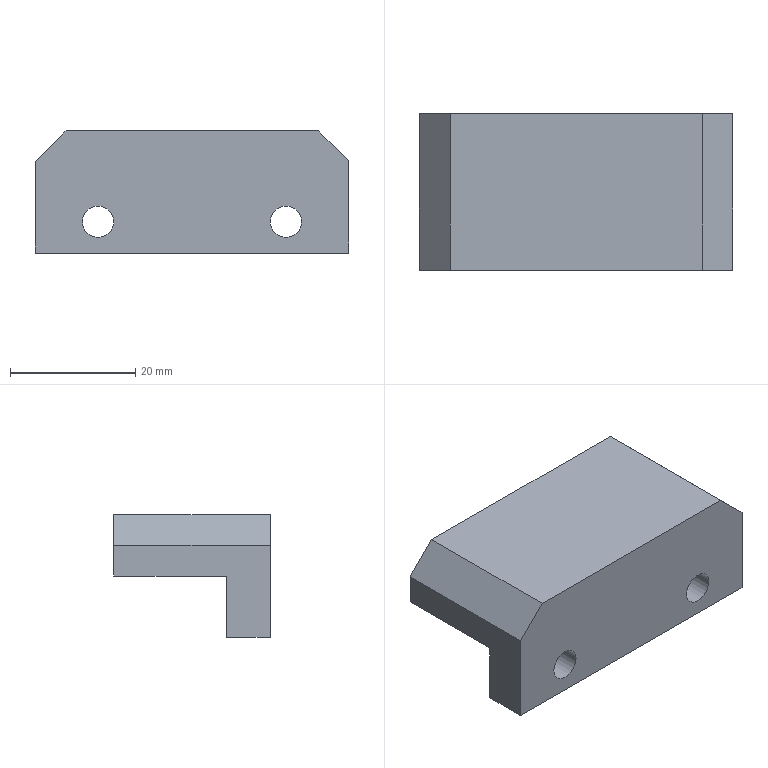Component | SolidWorks | LegSupport-1 | 1 solid | 22 faces | box 50 x 25 x 19.5 mm | volume 14508 mm3 | plane 10 | cylinder 8 | cone 4 | commonest cylinder face diameters 5 x4 2.5 x4
build123d program:
from build123d import *

# Parameters (mm, degrees)
SKETCH2_W             = 17
SKETCH2_H             = 50
BOSS_EXTRUDE1_DEPTH   = 25
M3_TAPPED_HOLE1_D     = 2.5
M3_TAPPED_HOLE1_DEPTH = 12.5
M3_TAPPED_HOLE1_TIP   = 0.7511
SKETCH5_W             = 10
SKETCH5_H             = 50
BOSS_EXTRUDE2_DEPTH   = 25
CUT_EXTRUDE1_DEPTH    = 18
SKETCH7_R             = 2.5
CUT_EXTRUDE2_DEPTH    = 38.027
CUT_EXTRUDE3_REACH    = 39.027


with BuildPart() as part:
    # Sketch2 → Boss-Extrude1 (new body)
    with BuildSketch(Plane(origin=(0, 0, 0), x_dir=(1, 0, 0), z_dir=(0, 1, 0))):
        Rectangle(SKETCH2_W, SKETCH2_H)
    extrude(amount=BOSS_EXTRUDE1_DEPTH)

    # M3 Tapped Hole1
    with Locations(Plane(origin=(6, 25, -15), x_dir=(0, 0, 1), z_dir=(0, 1, 0))):
        with Locations((0, 0), (30, 0)):
            Hole(M3_TAPPED_HOLE1_D / 2, depth=M3_TAPPED_HOLE1_DEPTH)
            with Locations((0, 0, -(M3_TAPPED_HOLE1_DEPTH + M3_TAPPED_HOLE1_TIP / 2))):  # 118° drill point
                Cone(0, M3_TAPPED_HOLE1_D / 2, M3_TAPPED_HOLE1_TIP, mode=Mode.SUBTRACT)

    # Sketch5 → Boss-Extrude2 (add)
    with BuildSketch(Plane(origin=(0, 25, 0), x_dir=(1, 0, 0), z_dir=(0, 1, 0))):
        with Locations((-6, 0)):
            Rectangle(SKETCH5_W, SKETCH5_H)
    extrude(amount=-BOSS_EXTRUDE2_DEPTH)

    # Sketch6 → Cut-Extrude1 (cut)
    with BuildSketch(Plane(origin=(0, 25, 0), x_dir=(1, 0, 0), z_dir=(0, 1, 0))):
        Polygon((-11, 25), (-1, 25), (-1.25, -25), (-11, -25), align=None)
    extrude(amount=-CUT_EXTRUDE1_DEPTH, mode=Mode.SUBTRACT)

    # Sketch7 → Cut-Extrude2 (cut, through all)
    with BuildSketch(Plane(origin=(0, 25, 0), x_dir=(1, 0, 0), z_dir=(0, 1, 0))):
        with Locations(Location((-6, 15, 0), (0, 0, 270))):
            Circle(SKETCH7_R)
        with Locations(Location((-6, -15, 0), (0, 0, 270))):
            Circle(SKETCH7_R)
    extrude(amount=-CUT_EXTRUDE2_DEPTH, mode=Mode.SUBTRACT)

    # Sketch8 → Cut-Extrude3 (cut, up to next)
    with BuildSketch(Plane(origin=(0, 25, 0), x_dir=(1, 0, 0), z_dir=(0, 1, 0)), mode=Mode.PRIVATE) as cut_extrude3_sk1:
        Polygon((8.5, 25), (3.75, 25), (8.5, 20.25), align=None)
    cut_extrude3_tool1 = extrude(cut_extrude3_sk1.sketch, amount=-CUT_EXTRUDE3_REACH, mode=Mode.PRIVATE) & part.part
    # Sketch8 → Cut-Extrude3 (cut, up to next)
    with BuildSketch(Plane(origin=(0, 25, 0), x_dir=(1, 0, 0), z_dir=(0, 1, 0)), mode=Mode.PRIVATE) as cut_extrude3_sk2:
        Polygon((8.5, -25), (8.5, -20.125), (3.625, -25), align=None)
    cut_extrude3_tool2 = extrude(cut_extrude3_sk2.sketch, amount=-CUT_EXTRUDE3_REACH, mode=Mode.PRIVATE) & part.part
    add(cut_extrude3_tool1.solids().sort_by_distance((6.917, 25, -23.417))[0], mode=Mode.SUBTRACT)
    add(cut_extrude3_tool2.solids().sort_by_distance((6.875, 25, 23.375))[0], mode=Mode.SUBTRACT)


solid = part.part

# Placed as in the assembly
solid = solid.moved(Location((-24.154, 53.266, -195.507), (0, -90, 0)))
STEP:
#1=CARTESIAN_POINT('',(-1.443,2.097,-7.933));
#2=VERTEX_POINT('',#1);
#3=CARTESIAN_POINT('',(-1.64,2.097,-7.933));
#4=VERTEX_POINT('',#3);
#5=CARTESIAN_POINT('',(-1.542,2.097,-7.933));
#6=DIRECTION('',(0.,1.,0.));
#7=DIRECTION('',(-1.,0.,0.));
#8=AXIS2_PLACEMENT_3D('',#5,#6,#7);
#9=CIRCLE('',#8,0.09843);
#10=EDGE_CURVE('',#2,#4,#9,.T.);
#11=ORIENTED_EDGE('',*,*,#10,.F.);
#12=CARTESIAN_POINT('',(-1.443,2.373,-7.933));
#13=VERTEX_POINT('',#12);
#14=CARTESIAN_POINT('',(-1.443,2.097,-7.933));
#15=DIRECTION('',(0.,1.,0.));
#16=VECTOR('',#15,39.37);
#17=LINE('',#14,#16);
#18=EDGE_CURVE('',#2,#13,#17,.T.);
#19=ORIENTED_EDGE('',*,*,#18,.T.);
#20=CARTESIAN_POINT('',(-1.64,2.373,-7.933));
#21=VERTEX_POINT('',#20);
#22=CARTESIAN_POINT('',(-1.542,2.373,-7.933));
#23=DIRECTION('',(0.,1.,0.));
#24=DIRECTION('',(-1.,0.,0.));
#25=AXIS2_PLACEMENT_3D('',#22,#23,#24);
#26=CIRCLE('',#25,0.09843);
#27=EDGE_CURVE('',#13,#21,#26,.T.);
#28=ORIENTED_EDGE('',*,*,#27,.T.);
#29=CARTESIAN_POINT('',(-1.64,2.097,-7.933));
#30=DIRECTION('',(0.,1.,0.));
#31=VECTOR('',#30,39.37);
#32=LINE('',#29,#31);
#33=EDGE_CURVE('',#4,#21,#32,.T.);
#34=ORIENTED_EDGE('',*,*,#33,.F.);
#35=EDGE_LOOP('',(#11,#19,#28,#34));
#36=FACE_OUTER_BOUND('',#35,.T.);
#37=CARTESIAN_POINT('',(-1.542,2.097,-7.933));
#38=DIRECTION('',(0.,1.,0.));
#39=DIRECTION('',(-1.,0.,0.));
#40=AXIS2_PLACEMENT_3D('',#37,#38,#39);
#41=CYLINDRICAL_SURFACE('',#40,0.09843);
#42=ADVANCED_FACE('',(#36),#41,.F.);
#43=CARTESIAN_POINT('',(-0.262,2.097,-7.933));
#44=VERTEX_POINT('',#43);
#45=CARTESIAN_POINT('',(-0.4588,2.097,-7.933));
#46=VERTEX_POINT('',#45);
#47=CARTESIAN_POINT('',(-0.3604,2.097,-7.933));
#48=DIRECTION('',(0.,1.,0.));
#49=DIRECTION('',(-1.,0.,0.));
#50=AXIS2_PLACEMENT_3D('',#47,#48,#49);
#51=CIRCLE('',#50,0.09843);
#52=EDGE_CURVE('',#44,#46,#51,.T.);
#53=ORIENTED_EDGE('',*,*,#52,.F.);
#54=CARTESIAN_POINT('',(-0.262,2.373,-7.933));
#55=VERTEX_POINT('',#54);
#56=CARTESIAN_POINT('',(-0.262,2.097,-7.933));
#57=DIRECTION('',(0.,1.,0.));
#58=VECTOR('',#57,39.37);
#59=LINE('',#56,#58);
#60=EDGE_CURVE('',#44,#55,#59,.T.);
#61=ORIENTED_EDGE('',*,*,#60,.T.);
#62=CARTESIAN_POINT('',(-0.4588,2.373,-7.933));
#63=VERTEX_POINT('',#62);
#64=CARTESIAN_POINT('',(-0.3604,2.373,-7.933));
#65=DIRECTION('',(0.,1.,0.));
#66=DIRECTION('',(-1.,0.,0.));
#67=AXIS2_PLACEMENT_3D('',#64,#65,#66);
#68=CIRCLE('',#67,0.09843);
#69=EDGE_CURVE('',#55,#63,#68,.T.);
#70=ORIENTED_EDGE('',*,*,#69,.T.);
#71=CARTESIAN_POINT('',(-0.4588,2.097,-7.933));
#72=DIRECTION('',(0.,1.,0.));
#73=VECTOR('',#72,39.37);
#74=LINE('',#71,#73);
#75=EDGE_CURVE('',#46,#63,#74,.T.);
#76=ORIENTED_EDGE('',*,*,#75,.F.);
#77=EDGE_LOOP('',(#53,#61,#70,#76));
#78=FACE_OUTER_BOUND('',#77,.T.);
#79=CARTESIAN_POINT('',(-0.3604,2.097,-7.933));
#80=DIRECTION('',(0.,1.,0.));
#81=DIRECTION('',(-1.,0.,0.));
#82=AXIS2_PLACEMENT_3D('',#79,#80,#81);
#83=CYLINDRICAL_SURFACE('',#82,0.09843);
#84=ADVANCED_FACE('',(#78),#83,.F.);
#85=CARTESIAN_POINT('',(-0.3112,2.589,-7.461));
#86=VERTEX_POINT('',#85);
#87=CARTESIAN_POINT('',(-0.4096,2.589,-7.461));
#88=VERTEX_POINT('',#87);
#89=CARTESIAN_POINT('',(-0.3604,2.589,-7.461));
#90=DIRECTION('',(0.,1.,0.));
#91=DIRECTION('',(-1.,0.,0.));
#92=AXIS2_PLACEMENT_3D('',#89,#90,#91);
#93=CIRCLE('',#92,0.04921);
#94=EDGE_CURVE('',#86,#88,#93,.T.);
#95=ORIENTED_EDGE('',*,*,#94,.F.);
#96=CARTESIAN_POINT('',(-0.3112,3.081,-7.461));
#97=VERTEX_POINT('',#96);
#98=CARTESIAN_POINT('',(-0.3112,3.081,-7.461));
#99=DIRECTION('',(0.,1.,0.));
#100=VECTOR('',#99,39.37);
#101=LINE('',#98,#100);
#102=EDGE_CURVE('',#86,#97,#101,.T.);
#103=ORIENTED_EDGE('',*,*,#102,.T.);
#104=CARTESIAN_POINT('',(-0.4096,3.081,-7.461));
#105=VERTEX_POINT('',#104);
#106=CARTESIAN_POINT('',(-0.3604,3.081,-7.461));
#107=DIRECTION('',(0.,1.,0.));
#108=DIRECTION('',(-1.,0.,0.));
#109=AXIS2_PLACEMENT_3D('',#106,#107,#108);
#110=CIRCLE('',#109,0.04921);
#111=EDGE_CURVE('',#97,#105,#110,.T.);
#112=ORIENTED_EDGE('',*,*,#111,.T.);
#113=CARTESIAN_POINT('',(-0.4096,3.081,-7.461));
#114=DIRECTION('',(0.,1.,0.));
#115=VECTOR('',#114,39.37);
#116=LINE('',#113,#115);
#117=EDGE_CURVE('',#88,#105,#116,.T.);
#118=ORIENTED_EDGE('',*,*,#117,.F.);
#119=EDGE_LOOP('',(#95,#103,#112,#118));
#120=FACE_OUTER_BOUND('',#119,.T.);
#121=CARTESIAN_POINT('',(-0.3604,3.081,-7.461));
#122=DIRECTION('',(0.,1.,0.));
#123=DIRECTION('',(-1.,0.,0.));
#124=AXIS2_PLACEMENT_3D('',#121,#122,#123);
#125=CYLINDRICAL_SURFACE('',#124,0.04921);
#126=ADVANCED_FACE('',(#120),#125,.F.);
#127=CARTESIAN_POINT('',(-0.3604,2.56,-7.461));
#128=VERTEX_POINT('',#127);
#129=CARTESIAN_POINT('',(-0.4096,2.589,-7.461));
#130=DIRECTION('',(-0.8572,0.515,-0.));
#131=VECTOR('',#130,39.37);
#132=LINE('',#129,#131);
#133=EDGE_CURVE('',#128,#88,#132,.T.);
#134=ORIENTED_EDGE('',*,*,#133,.F.);
#135=CARTESIAN_POINT('',(-0.3112,2.589,-7.461));
#136=DIRECTION('',(0.8572,0.515,0.));
#137=VECTOR('',#136,39.37);
#138=LINE('',#135,#137);
#139=EDGE_CURVE('',#128,#86,#138,.T.);
#140=ORIENTED_EDGE('',*,*,#139,.T.);
#141=ORIENTED_EDGE('',*,*,#94,.T.);
#142=EDGE_LOOP('',(#134,#140,#141));
#143=FACE_OUTER_BOUND('',#142,.T.);
#144=CARTESIAN_POINT('',(-0.3604,2.589,-7.461));
#145=DIRECTION('',(0.,1.,0.));
#146=DIRECTION('',(-1.,0.,0.));
#147=AXIS2_PLACEMENT_3D('',#144,#145,#146);
#148=CONICAL_SURFACE('',#147,0.04921,1.03);
#149=ADVANCED_FACE('',(#143),#148,.F.);
#150=CARTESIAN_POINT('',(-1.492,2.589,-7.461));
#151=VERTEX_POINT('',#150);
#152=CARTESIAN_POINT('',(-1.591,2.589,-7.461));
#153=VERTEX_POINT('',#152);
#154=CARTESIAN_POINT('',(-1.542,2.589,-7.461));
#155=DIRECTION('',(0.,1.,0.));
#156=DIRECTION('',(-1.,0.,0.));
#157=AXIS2_PLACEMENT_3D('',#154,#155,#156);
#158=CIRCLE('',#157,0.04921);
#159=EDGE_CURVE('',#151,#153,#158,.T.);
#160=ORIENTED_EDGE('',*,*,#159,.F.);
#161=CARTESIAN_POINT('',(-1.492,3.081,-7.461));
#162=VERTEX_POINT('',#161);
#163=CARTESIAN_POINT('',(-1.492,3.081,-7.461));
#164=DIRECTION('',(0.,1.,0.));
#165=VECTOR('',#164,39.37);
#166=LINE('',#163,#165);
#167=EDGE_CURVE('',#151,#162,#166,.T.);
#168=ORIENTED_EDGE('',*,*,#167,.T.);
#169=CARTESIAN_POINT('',(-1.591,3.081,-7.461));
#170=VERTEX_POINT('',#169);
#171=CARTESIAN_POINT('',(-1.542,3.081,-7.461));
#172=DIRECTION('',(0.,1.,0.));
#173=DIRECTION('',(-1.,0.,0.));
#174=AXIS2_PLACEMENT_3D('',#171,#172,#173);
#175=CIRCLE('',#174,0.04921);
#176=EDGE_CURVE('',#162,#170,#175,.T.);
#177=ORIENTED_EDGE('',*,*,#176,.T.);
#178=CARTESIAN_POINT('',(-1.591,3.081,-7.461));
#179=DIRECTION('',(0.,1.,0.));
#180=VECTOR('',#179,39.37);
#181=LINE('',#178,#180);
#182=EDGE_CURVE('',#153,#170,#181,.T.);
#183=ORIENTED_EDGE('',*,*,#182,.F.);
#184=EDGE_LOOP('',(#160,#168,#177,#183));
#185=FACE_OUTER_BOUND('',#184,.T.);
#186=CARTESIAN_POINT('',(-1.542,3.081,-7.461));
#187=DIRECTION('',(0.,1.,0.));
#188=DIRECTION('',(-1.,0.,0.));
#189=AXIS2_PLACEMENT_3D('',#186,#187,#188);
#190=CYLINDRICAL_SURFACE('',#189,0.04921);
#191=ADVANCED_FACE('',(#185),#190,.F.);
#192=CARTESIAN_POINT('',(-1.542,2.56,-7.461));
#193=VERTEX_POINT('',#192);
#194=CARTESIAN_POINT('',(-1.591,2.589,-7.461));
#195=DIRECTION('',(-0.8572,0.515,-0.));
#196=VECTOR('',#195,39.37);
#197=LINE('',#194,#196);
#198=EDGE_CURVE('',#193,#153,#197,.T.);
#199=ORIENTED_EDGE('',*,*,#198,.F.);
#200=CARTESIAN_POINT('',(-1.492,2.589,-7.461));
#201=DIRECTION('',(0.8572,0.515,0.));
#202=VECTOR('',#201,39.37);
#203=LINE('',#200,#202);
#204=EDGE_CURVE('',#193,#151,#203,.T.);
#205=ORIENTED_EDGE('',*,*,#204,.T.);
#206=ORIENTED_EDGE('',*,*,#159,.T.);
#207=EDGE_LOOP('',(#199,#205,#206));
#208=FACE_OUTER_BOUND('',#207,.T.);
#209=CARTESIAN_POINT('',(-1.542,2.589,-7.461));
#210=DIRECTION('',(0.,1.,0.));
#211=DIRECTION('',(-1.,0.,0.));
#212=AXIS2_PLACEMENT_3D('',#209,#210,#211);
#213=CONICAL_SURFACE('',#212,0.04921,1.03);
#214=ADVANCED_FACE('',(#208),#213,.F.);
#215=CARTESIAN_POINT('',(-1.743,2.097,-7.362));
#216=VERTEX_POINT('',#215);
#217=CARTESIAN_POINT('',(-1.743,3.081,-7.362));
#218=VERTEX_POINT('',#217);
#219=CARTESIAN_POINT('',(-1.743,2.097,-7.362));
#220=DIRECTION('',(0.,1.,0.));
#221=VECTOR('',#220,39.37);
#222=LINE('',#219,#221);
#223=EDGE_CURVE('',#216,#218,#222,.T.);
#224=ORIENTED_EDGE('',*,*,#223,.F.);
#225=CARTESIAN_POINT('',(-0.1537,2.097,-7.362));
#226=VERTEX_POINT('',#225);
#227=CARTESIAN_POINT('',(0.03329,2.097,-7.362));
#228=DIRECTION('',(1.,0.,0.));
#229=VECTOR('',#228,39.37);
#230=LINE('',#227,#229);
#231=EDGE_CURVE('',#216,#226,#230,.T.);
#232=ORIENTED_EDGE('',*,*,#231,.T.);
#233=CARTESIAN_POINT('',(-0.1537,3.081,-7.362));
#234=VERTEX_POINT('',#233);
#235=CARTESIAN_POINT('',(-0.1537,2.097,-7.362));
#236=DIRECTION('',(0.,1.,0.));
#237=VECTOR('',#236,39.37);
#238=LINE('',#235,#237);
#239=EDGE_CURVE('',#226,#234,#238,.T.);
#240=ORIENTED_EDGE('',*,*,#239,.T.);
#241=CARTESIAN_POINT('',(0.03329,3.081,-7.362));
#242=DIRECTION('',(1.,0.,0.));
#243=VECTOR('',#242,39.37);
#244=LINE('',#241,#243);
#245=EDGE_CURVE('',#218,#234,#244,.T.);
#246=ORIENTED_EDGE('',*,*,#245,.F.);
#247=EDGE_LOOP('',(#224,#232,#240,#246));
#248=FACE_OUTER_BOUND('',#247,.T.);
#249=CARTESIAN_POINT('',(0.03329,3.081,-7.362));
#250=DIRECTION('',(0.,0.,-1.));
#251=DIRECTION('',(-1.,0.,-0.));
#252=AXIS2_PLACEMENT_3D('',#249,#250,#251);
#253=PLANE('',#252);
#254=ADVANCED_FACE('',(#248),#253,.F.);
#255=CARTESIAN_POINT('',(-1.935,2.097,-7.554));
#256=VERTEX_POINT('',#255);
#257=CARTESIAN_POINT('',(-1.935,3.081,-7.554));
#258=VERTEX_POINT('',#257);
#259=CARTESIAN_POINT('',(-1.935,2.097,-7.554));
#260=DIRECTION('',(0.,1.,0.));
#261=VECTOR('',#260,39.37);
#262=LINE('',#259,#261);
#263=EDGE_CURVE('',#256,#258,#262,.T.);
#264=ORIENTED_EDGE('',*,*,#263,.T.);
#265=CARTESIAN_POINT('',(-1.935,3.081,-7.746));
#266=VERTEX_POINT('',#265);
#267=CARTESIAN_POINT('',(-1.935,3.081,-8.032));
#268=DIRECTION('',(-0.,0.,1.));
#269=VECTOR('',#268,39.37);
#270=LINE('',#267,#269);
#271=EDGE_CURVE('',#266,#258,#270,.T.);
#272=ORIENTED_EDGE('',*,*,#271,.F.);
#273=CARTESIAN_POINT('',(-1.935,2.373,-7.746));
#274=VERTEX_POINT('',#273);
#275=CARTESIAN_POINT('',(-1.935,2.373,-7.746));
#276=DIRECTION('',(0.,1.,0.));
#277=VECTOR('',#276,39.37);
#278=LINE('',#275,#277);
#279=EDGE_CURVE('',#274,#266,#278,.T.);
#280=ORIENTED_EDGE('',*,*,#279,.F.);
#281=CARTESIAN_POINT('',(-1.935,2.373,-8.13));
#282=VERTEX_POINT('',#281);
#283=CARTESIAN_POINT('',(-1.935,2.373,-8.13));
#284=DIRECTION('',(0.,0.,1.));
#285=VECTOR('',#284,39.37);
#286=LINE('',#283,#285);
#287=EDGE_CURVE('',#282,#274,#286,.T.);
#288=ORIENTED_EDGE('',*,*,#287,.F.);
#289=CARTESIAN_POINT('',(-1.935,2.097,-8.13));
#290=VERTEX_POINT('',#289);
#291=CARTESIAN_POINT('',(-1.935,2.097,-8.13));
#292=DIRECTION('',(0.,1.,0.));
#293=VECTOR('',#292,39.37);
#294=LINE('',#291,#293);
#295=EDGE_CURVE('',#290,#282,#294,.T.);
#296=ORIENTED_EDGE('',*,*,#295,.F.);
#297=CARTESIAN_POINT('',(-1.935,2.097,-8.032));
#298=DIRECTION('',(-0.,0.,1.));
#299=VECTOR('',#298,39.37);
#300=LINE('',#297,#299);
#301=EDGE_CURVE('',#290,#256,#300,.T.);
#302=ORIENTED_EDGE('',*,*,#301,.T.);
#303=EDGE_LOOP('',(#264,#272,#280,#288,#296,#302));
#304=FACE_OUTER_BOUND('',#303,.T.);
#305=CARTESIAN_POINT('',(-1.935,3.081,-8.032));
#306=DIRECTION('',(1.,0.,0.));
#307=DIRECTION('',(0.,0.,-1.));
#308=AXIS2_PLACEMENT_3D('',#305,#306,#307);
#309=PLANE('',#308);
#310=ADVANCED_FACE('',(#304),#309,.F.);
#311=CARTESIAN_POINT('',(-0.3604,3.081,-7.461));
#312=DIRECTION('',(0.,1.,0.));
#313=DIRECTION('',(-1.,0.,0.));
#314=AXIS2_PLACEMENT_3D('',#311,#312,#313);
#315=CIRCLE('',#314,0.04921);
#316=EDGE_CURVE('',#105,#97,#315,.T.);
#317=ORIENTED_EDGE('',*,*,#316,.F.);
#318=ORIENTED_EDGE('',*,*,#111,.F.);
#319=EDGE_LOOP('',(#317,#318));
#320=FACE_BOUND('',#319,.T.);
#321=CARTESIAN_POINT('',(-1.542,3.081,-7.461));
#322=DIRECTION('',(0.,1.,0.));
#323=DIRECTION('',(-1.,0.,0.));
#324=AXIS2_PLACEMENT_3D('',#321,#322,#323);
#325=CIRCLE('',#324,0.04921);
#326=EDGE_CURVE('',#170,#162,#325,.T.);
#327=ORIENTED_EDGE('',*,*,#326,.F.);
#328=ORIENTED_EDGE('',*,*,#176,.F.);
#329=EDGE_LOOP('',(#327,#328));
#330=FACE_BOUND('',#329,.T.);
#331=ORIENTED_EDGE('',*,*,#271,.T.);
#332=CARTESIAN_POINT('',(-1.514,3.081,-7.134));
#333=DIRECTION('',(0.7071,0.,0.7071));
#334=VECTOR('',#333,39.37);
#335=LINE('',#332,#334);
#336=EDGE_CURVE('',#258,#218,#335,.T.);
#337=ORIENTED_EDGE('',*,*,#336,.T.);
#338=ORIENTED_EDGE('',*,*,#245,.T.);
#339=CARTESIAN_POINT('',(0.03329,3.081,-7.549));
#340=VERTEX_POINT('',#339);
#341=CARTESIAN_POINT('',(-0.385,3.081,-7.131));
#342=DIRECTION('',(-0.7071,0.,0.7071));
#343=VECTOR('',#342,39.37);
#344=LINE('',#341,#343);
#345=EDGE_CURVE('',#340,#234,#344,.T.);
#346=ORIENTED_EDGE('',*,*,#345,.F.);
#347=CARTESIAN_POINT('',(0.03329,3.081,-7.736));
#348=VERTEX_POINT('',#347);
#349=CARTESIAN_POINT('',(0.03329,3.081,-8.032));
#350=DIRECTION('',(0.,0.,-1.));
#351=VECTOR('',#350,39.37);
#352=LINE('',#349,#351);
#353=EDGE_CURVE('',#340,#348,#352,.T.);
#354=ORIENTED_EDGE('',*,*,#353,.T.);
#355=CARTESIAN_POINT('',(0.03329,3.081,-7.736));
#356=DIRECTION('',(1.,0.,0.005));
#357=VECTOR('',#356,39.37);
#358=LINE('',#355,#357);
#359=EDGE_CURVE('',#266,#348,#358,.T.);
#360=ORIENTED_EDGE('',*,*,#359,.F.);
#361=EDGE_LOOP('',(#331,#337,#338,#346,#354,#360));
#362=FACE_OUTER_BOUND('',#361,.T.);
#363=CARTESIAN_POINT('',(-0.951,3.081,-7.697));
#364=DIRECTION('',(0.,1.,0.));
#365=DIRECTION('',(-1.,0.,-0.));
#366=AXIS2_PLACEMENT_3D('',#363,#364,#365);
#367=PLANE('',#366);
#368=ADVANCED_FACE('',(#320,#330,#362),#367,.T.);
#369=CARTESIAN_POINT('',(-0.3604,2.097,-7.933));
#370=DIRECTION('',(0.,1.,0.));
#371=DIRECTION('',(-1.,0.,0.));
#372=AXIS2_PLACEMENT_3D('',#369,#370,#371);
#373=CIRCLE('',#372,0.09843);
#374=EDGE_CURVE('',#46,#44,#373,.T.);
#375=ORIENTED_EDGE('',*,*,#374,.T.);
#376=ORIENTED_EDGE('',*,*,#52,.T.);
#377=EDGE_LOOP('',(#375,#376));
#378=FACE_BOUND('',#377,.T.);
#379=CARTESIAN_POINT('',(-1.542,2.097,-7.933));
#380=DIRECTION('',(0.,1.,0.));
#381=DIRECTION('',(-1.,0.,0.));
#382=AXIS2_PLACEMENT_3D('',#379,#380,#381);
#383=CIRCLE('',#382,0.09843);
#384=EDGE_CURVE('',#4,#2,#383,.T.);
#385=ORIENTED_EDGE('',*,*,#384,.T.);
#386=ORIENTED_EDGE('',*,*,#10,.T.);
#387=EDGE_LOOP('',(#385,#386));
#388=FACE_BOUND('',#387,.T.);
#389=CARTESIAN_POINT('',(-1.514,2.097,-7.134));
#390=DIRECTION('',(-0.7071,0.,-0.7071));
#391=VECTOR('',#390,39.37);
#392=LINE('',#389,#391);
#393=EDGE_CURVE('',#216,#256,#392,.T.);
#394=ORIENTED_EDGE('',*,*,#393,.T.);
#395=ORIENTED_EDGE('',*,*,#301,.F.);
#396=CARTESIAN_POINT('',(0.03329,2.097,-8.13));
#397=VERTEX_POINT('',#396);
#398=CARTESIAN_POINT('',(0.03329,2.097,-8.13));
#399=DIRECTION('',(-1.,0.,-0.));
#400=VECTOR('',#399,39.37);
#401=LINE('',#398,#400);
#402=EDGE_CURVE('',#397,#290,#401,.T.);
#403=ORIENTED_EDGE('',*,*,#402,.F.);
#404=CARTESIAN_POINT('',(0.03329,2.097,-7.549));
#405=VERTEX_POINT('',#404);
#406=CARTESIAN_POINT('',(0.03329,2.097,-8.032));
#407=DIRECTION('',(0.,0.,-1.));
#408=VECTOR('',#407,39.37);
#409=LINE('',#406,#408);
#410=EDGE_CURVE('',#405,#397,#409,.T.);
#411=ORIENTED_EDGE('',*,*,#410,.F.);
#412=CARTESIAN_POINT('',(-0.385,2.097,-7.131));
#413=DIRECTION('',(0.7071,0.,-0.7071));
#414=VECTOR('',#413,39.37);
#415=LINE('',#412,#414);
#416=EDGE_CURVE('',#226,#405,#415,.T.);
#417=ORIENTED_EDGE('',*,*,#416,.F.);
#418=ORIENTED_EDGE('',*,*,#231,.F.);
#419=EDGE_LOOP('',(#394,#395,#403,#411,#417,#418));
#420=FACE_OUTER_BOUND('',#419,.T.);
#421=CARTESIAN_POINT('',(-0.951,2.097,-7.697));
#422=DIRECTION('',(0.,1.,0.));
#423=DIRECTION('',(-1.,0.,-0.));
#424=AXIS2_PLACEMENT_3D('',#421,#422,#423);
#425=PLANE('',#424);
#426=ADVANCED_FACE('',(#378,#388,#420),#425,.F.);
#427=ORIENTED_EDGE('',*,*,#295,.T.);
#428=CARTESIAN_POINT('',(0.03329,2.373,-8.13));
#429=VERTEX_POINT('',#428);
#430=CARTESIAN_POINT('',(0.03329,2.373,-8.13));
#431=DIRECTION('',(-1.,0.,-0.));
#432=VECTOR('',#431,39.37);
#433=LINE('',#430,#432);
#434=EDGE_CURVE('',#429,#282,#433,.T.);
#435=ORIENTED_EDGE('',*,*,#434,.F.);
#436=CARTESIAN_POINT('',(0.03329,2.097,-8.13));
#437=DIRECTION('',(0.,1.,0.));
#438=VECTOR('',#437,39.37);
#439=LINE('',#436,#438);
#440=EDGE_CURVE('',#397,#429,#439,.T.);
#441=ORIENTED_EDGE('',*,*,#440,.F.);
#442=ORIENTED_EDGE('',*,*,#402,.T.);
#443=EDGE_LOOP('',(#427,#435,#441,#442));
#444=FACE_OUTER_BOUND('',#443,.T.);
#445=CARTESIAN_POINT('',(0.03329,2.097,-8.13));
#446=DIRECTION('',(0.,0.,-1.));
#447=DIRECTION('',(-1.,0.,-0.));
#448=AXIS2_PLACEMENT_3D('',#445,#446,#447);
#449=PLANE('',#448);
#450=ADVANCED_FACE('',(#444),#449,.T.);
#451=ORIENTED_EDGE('',*,*,#353,.F.);
#452=CARTESIAN_POINT('',(0.03329,2.097,-7.549));
#453=DIRECTION('',(0.,1.,0.));
#454=VECTOR('',#453,39.37);
#455=LINE('',#452,#454);
#456=EDGE_CURVE('',#405,#340,#455,.T.);
#457=ORIENTED_EDGE('',*,*,#456,.F.);
#458=ORIENTED_EDGE('',*,*,#410,.T.);
#459=ORIENTED_EDGE('',*,*,#440,.T.);
#460=CARTESIAN_POINT('',(0.03329,2.373,-7.736));
#461=VERTEX_POINT('',#460);
#462=CARTESIAN_POINT('',(0.03329,2.373,-8.13));
#463=DIRECTION('',(-0.,0.,-1.));
#464=VECTOR('',#463,39.37);
#465=LINE('',#462,#464);
#466=EDGE_CURVE('',#461,#429,#465,.T.);
#467=ORIENTED_EDGE('',*,*,#466,.F.);
#468=CARTESIAN_POINT('',(0.03329,2.373,-7.736));
#469=DIRECTION('',(0.,1.,0.));
#470=VECTOR('',#469,39.37);
#471=LINE('',#468,#470);
#472=EDGE_CURVE('',#461,#348,#471,.T.);
#473=ORIENTED_EDGE('',*,*,#472,.T.);
#474=EDGE_LOOP('',(#451,#457,#458,#459,#467,#473));
#475=FACE_OUTER_BOUND('',#474,.T.);
#476=CARTESIAN_POINT('',(0.03329,3.081,-8.032));
#477=DIRECTION('',(-1.,0.,-0.));
#478=DIRECTION('',(-0.,0.,1.));
#479=AXIS2_PLACEMENT_3D('',#476,#477,#478);
#480=PLANE('',#479);
#481=ADVANCED_FACE('',(#475),#480,.F.);
#482=ORIENTED_EDGE('',*,*,#204,.F.);
#483=ORIENTED_EDGE('',*,*,#198,.T.);
#484=CARTESIAN_POINT('',(-1.542,2.589,-7.461));
#485=DIRECTION('',(0.,1.,0.));
#486=DIRECTION('',(-1.,0.,0.));
#487=AXIS2_PLACEMENT_3D('',#484,#485,#486);
#488=CIRCLE('',#487,0.04921);
#489=EDGE_CURVE('',#153,#151,#488,.T.);
#490=ORIENTED_EDGE('',*,*,#489,.T.);
#491=EDGE_LOOP('',(#482,#483,#490));
#492=FACE_OUTER_BOUND('',#491,.T.);
#493=CARTESIAN_POINT('',(-1.542,2.589,-7.461));
#494=DIRECTION('',(0.,1.,0.));
#495=DIRECTION('',(-1.,0.,0.));
#496=AXIS2_PLACEMENT_3D('',#493,#494,#495);
#497=CONICAL_SURFACE('',#496,0.04921,1.03);
#498=ADVANCED_FACE('',(#492),#497,.F.);
#499=ORIENTED_EDGE('',*,*,#167,.F.);
#500=ORIENTED_EDGE('',*,*,#489,.F.);
#501=ORIENTED_EDGE('',*,*,#182,.T.);
#502=ORIENTED_EDGE('',*,*,#326,.T.);
#503=EDGE_LOOP('',(#499,#500,#501,#502));
#504=FACE_OUTER_BOUND('',#503,.T.);
#505=CARTESIAN_POINT('',(-1.542,3.081,-7.461));
#506=DIRECTION('',(0.,1.,0.));
#507=DIRECTION('',(-1.,0.,0.));
#508=AXIS2_PLACEMENT_3D('',#505,#506,#507);
#509=CYLINDRICAL_SURFACE('',#508,0.04921);
#510=ADVANCED_FACE('',(#504),#509,.F.);
#511=ORIENTED_EDGE('',*,*,#139,.F.);
#512=ORIENTED_EDGE('',*,*,#133,.T.);
#513=CARTESIAN_POINT('',(-0.3604,2.589,-7.461));
#514=DIRECTION('',(0.,1.,0.));
#515=DIRECTION('',(-1.,0.,0.));
#516=AXIS2_PLACEMENT_3D('',#513,#514,#515);
#517=CIRCLE('',#516,0.04921);
#518=EDGE_CURVE('',#88,#86,#517,.T.);
#519=ORIENTED_EDGE('',*,*,#518,.T.);
#520=EDGE_LOOP('',(#511,#512,#519));
#521=FACE_OUTER_BOUND('',#520,.T.);
#522=CARTESIAN_POINT('',(-0.3604,2.589,-7.461));
#523=DIRECTION('',(0.,1.,0.));
#524=DIRECTION('',(-1.,0.,0.));
#525=AXIS2_PLACEMENT_3D('',#522,#523,#524);
#526=CONICAL_SURFACE('',#525,0.04921,1.03);
#527=ADVANCED_FACE('',(#521),#526,.F.);
#528=ORIENTED_EDGE('',*,*,#102,.F.);
#529=ORIENTED_EDGE('',*,*,#518,.F.);
#530=ORIENTED_EDGE('',*,*,#117,.T.);
#531=ORIENTED_EDGE('',*,*,#316,.T.);
#532=EDGE_LOOP('',(#528,#529,#530,#531));
#533=FACE_OUTER_BOUND('',#532,.T.);
#534=CARTESIAN_POINT('',(-0.3604,3.081,-7.461));
#535=DIRECTION('',(0.,1.,0.));
#536=DIRECTION('',(-1.,0.,0.));
#537=AXIS2_PLACEMENT_3D('',#534,#535,#536);
#538=CYLINDRICAL_SURFACE('',#537,0.04921);
#539=ADVANCED_FACE('',(#533),#538,.F.);
#540=ORIENTED_EDGE('',*,*,#359,.T.);
#541=ORIENTED_EDGE('',*,*,#472,.F.);
#542=CARTESIAN_POINT('',(0.03329,2.373,-7.736));
#543=DIRECTION('',(1.,0.,0.005));
#544=VECTOR('',#543,39.37);
#545=LINE('',#542,#544);
#546=EDGE_CURVE('',#274,#461,#545,.T.);
#547=ORIENTED_EDGE('',*,*,#546,.F.);
#548=ORIENTED_EDGE('',*,*,#279,.T.);
#549=EDGE_LOOP('',(#540,#541,#547,#548));
#550=FACE_OUTER_BOUND('',#549,.T.);
#551=CARTESIAN_POINT('',(0.03329,2.373,-7.736));
#552=DIRECTION('',(-0.005,0.,1.));
#553=DIRECTION('',(1.,0.,0.005));
#554=AXIS2_PLACEMENT_3D('',#551,#552,#553);
#555=PLANE('',#554);
#556=ADVANCED_FACE('',(#550),#555,.F.);
#557=CARTESIAN_POINT('',(-1.542,2.373,-7.933));
#558=DIRECTION('',(0.,1.,0.));
#559=DIRECTION('',(-1.,0.,0.));
#560=AXIS2_PLACEMENT_3D('',#557,#558,#559);
#561=CIRCLE('',#560,0.09843);
#562=EDGE_CURVE('',#21,#13,#561,.T.);
#563=ORIENTED_EDGE('',*,*,#562,.F.);
#564=ORIENTED_EDGE('',*,*,#27,.F.);
#565=EDGE_LOOP('',(#563,#564));
#566=FACE_BOUND('',#565,.T.);
#567=CARTESIAN_POINT('',(-0.3604,2.373,-7.933));
#568=DIRECTION('',(0.,1.,0.));
#569=DIRECTION('',(-1.,0.,0.));
#570=AXIS2_PLACEMENT_3D('',#567,#568,#569);
#571=CIRCLE('',#570,0.09843);
#572=EDGE_CURVE('',#63,#55,#571,.T.);
#573=ORIENTED_EDGE('',*,*,#572,.F.);
#574=ORIENTED_EDGE('',*,*,#69,.F.);
#575=EDGE_LOOP('',(#573,#574));
#576=FACE_BOUND('',#575,.T.);
#577=ORIENTED_EDGE('',*,*,#546,.T.);
#578=ORIENTED_EDGE('',*,*,#466,.T.);
#579=ORIENTED_EDGE('',*,*,#434,.T.);
#580=ORIENTED_EDGE('',*,*,#287,.T.);
#581=EDGE_LOOP('',(#577,#578,#579,#580));
#582=FACE_OUTER_BOUND('',#581,.T.);
#583=CARTESIAN_POINT('',(-0.951,2.373,-7.697));
#584=DIRECTION('',(0.,1.,0.));
#585=DIRECTION('',(-1.,0.,-0.));
#586=AXIS2_PLACEMENT_3D('',#583,#584,#585);
#587=PLANE('',#586);
#588=ADVANCED_FACE('',(#566,#576,#582),#587,.T.);
#589=ORIENTED_EDGE('',*,*,#60,.F.);
#590=ORIENTED_EDGE('',*,*,#374,.F.);
#591=ORIENTED_EDGE('',*,*,#75,.T.);
#592=ORIENTED_EDGE('',*,*,#572,.T.);
#593=EDGE_LOOP('',(#589,#590,#591,#592));
#594=FACE_OUTER_BOUND('',#593,.T.);
#595=CARTESIAN_POINT('',(-0.3604,2.097,-7.933));
#596=DIRECTION('',(0.,1.,0.));
#597=DIRECTION('',(-1.,0.,0.));
#598=AXIS2_PLACEMENT_3D('',#595,#596,#597);
#599=CYLINDRICAL_SURFACE('',#598,0.09843);
#600=ADVANCED_FACE('',(#594),#599,.F.);
#601=ORIENTED_EDGE('',*,*,#18,.F.);
#602=ORIENTED_EDGE('',*,*,#384,.F.);
#603=ORIENTED_EDGE('',*,*,#33,.T.);
#604=ORIENTED_EDGE('',*,*,#562,.T.);
#605=EDGE_LOOP('',(#601,#602,#603,#604));
#606=FACE_OUTER_BOUND('',#605,.T.);
#607=CARTESIAN_POINT('',(-1.542,2.097,-7.933));
#608=DIRECTION('',(0.,1.,0.));
#609=DIRECTION('',(-1.,0.,0.));
#610=AXIS2_PLACEMENT_3D('',#607,#608,#609);
#611=CYLINDRICAL_SURFACE('',#610,0.09843);
#612=ADVANCED_FACE('',(#606),#611,.F.);
#613=ORIENTED_EDGE('',*,*,#416,.T.);
#614=ORIENTED_EDGE('',*,*,#456,.T.);
#615=ORIENTED_EDGE('',*,*,#345,.T.);
#616=ORIENTED_EDGE('',*,*,#239,.F.);
#617=EDGE_LOOP('',(#613,#614,#615,#616));
#618=FACE_OUTER_BOUND('',#617,.T.);
#619=CARTESIAN_POINT('',(-0.385,2.097,-7.131));
#620=DIRECTION('',(-0.7071,0.,-0.7071));
#621=DIRECTION('',(-0.7071,0.,0.7071));
#622=AXIS2_PLACEMENT_3D('',#619,#620,#621);
#623=PLANE('',#622);
#624=ADVANCED_FACE('',(#618),#623,.F.);
#625=ORIENTED_EDGE('',*,*,#223,.T.);
#626=ORIENTED_EDGE('',*,*,#336,.F.);
#627=ORIENTED_EDGE('',*,*,#263,.F.);
#628=ORIENTED_EDGE('',*,*,#393,.F.);
#629=EDGE_LOOP('',(#625,#626,#627,#628));
#630=FACE_OUTER_BOUND('',#629,.T.);
#631=CARTESIAN_POINT('',(-1.514,2.097,-7.134));
#632=DIRECTION('',(-0.7071,0.,0.7071));
#633=DIRECTION('',(0.7071,0.,0.7071));
#634=AXIS2_PLACEMENT_3D('',#631,#632,#633);
#635=PLANE('',#634);
#636=ADVANCED_FACE('',(#630),#635,.T.);
#637=CLOSED_SHELL('',(#42,#84,#126,#149,#191,#214,#254,#310,#368,#426,#450,#481,#498,#510,#527,#539,#556,#588,#600,#612,#624,#636));
#638=MANIFOLD_SOLID_BREP('',#637);
#639=CARTESIAN_POINT('',(0.,0.,0.));
#640=DIRECTION('',(0.,0.,1.));
#641=DIRECTION('',(1.,0.,0.));
#642=AXIS2_PLACEMENT_3D('',#639,#640,#641);
#643=(LENGTH_UNIT()NAMED_UNIT(*)SI_UNIT($,.METRE.));
#644=LENGTH_MEASURE_WITH_UNIT(LENGTH_MEASURE(0.0254),#643);
#645=DIMENSIONAL_EXPONENTS(1.,0.,0.,0.,0.,0.,0.);
#646=(CONVERSION_BASED_UNIT('',#644)LENGTH_UNIT()NAMED_UNIT(#645));
#647=UNCERTAINTY_MEASURE_WITH_UNIT(LENGTH_MEASURE(0.00001),#646,'','');
#648=(NAMED_UNIT(*)PLANE_ANGLE_UNIT()SI_UNIT($,.RADIAN.));
#649=(NAMED_UNIT(*)SI_UNIT($,.STERADIAN.)SOLID_ANGLE_UNIT());
#650=(GEOMETRIC_REPRESENTATION_CONTEXT(3)GLOBAL_UNCERTAINTY_ASSIGNED_CONTEXT((#647))GLOBAL_UNIT_ASSIGNED_CONTEXT((#646,#648,#649))REPRESENTATION_CONTEXT('',''));
#651=ADVANCED_BREP_SHAPE_REPRESENTATION('',(#638,#642),#650);
#652=COLOUR_RGB('',0.7922,0.8196,0.9333);
#653=FILL_AREA_STYLE_COLOUR('',#652);
#654=FILL_AREA_STYLE('',(#653));
#655=SURFACE_STYLE_FILL_AREA(#654);
#656=SURFACE_SIDE_STYLE('',(#655));
#657=SURFACE_STYLE_USAGE(.BOTH.,#656);
#658=PRESENTATION_STYLE_ASSIGNMENT((#657));
#659=STYLED_ITEM('',(#658),#638);
#660=(LENGTH_UNIT()NAMED_UNIT(*)SI_UNIT($,.METRE.));
#661=LENGTH_MEASURE_WITH_UNIT(LENGTH_MEASURE(0.0254),#660);
#662=DIMENSIONAL_EXPONENTS(1.,0.,0.,0.,0.,0.,0.);
#663=(CONVERSION_BASED_UNIT('',#661)LENGTH_UNIT()NAMED_UNIT(#662));
#664=UNCERTAINTY_MEASURE_WITH_UNIT(LENGTH_MEASURE(0.00001),#663,'','');
#665=(NAMED_UNIT(*)PLANE_ANGLE_UNIT()SI_UNIT($,.RADIAN.));
#666=(NAMED_UNIT(*)SI_UNIT($,.STERADIAN.)SOLID_ANGLE_UNIT());
#667=(GEOMETRIC_REPRESENTATION_CONTEXT(3)GLOBAL_UNCERTAINTY_ASSIGNED_CONTEXT((#664))GLOBAL_UNIT_ASSIGNED_CONTEXT((#663,#665,#666))REPRESENTATION_CONTEXT('',''));
#668=MECHANICAL_DESIGN_GEOMETRIC_PRESENTATION_REPRESENTATION('',(#659),#667);
#669=PRESENTATION_LAYER_ASSIGNMENT('','',(#659));